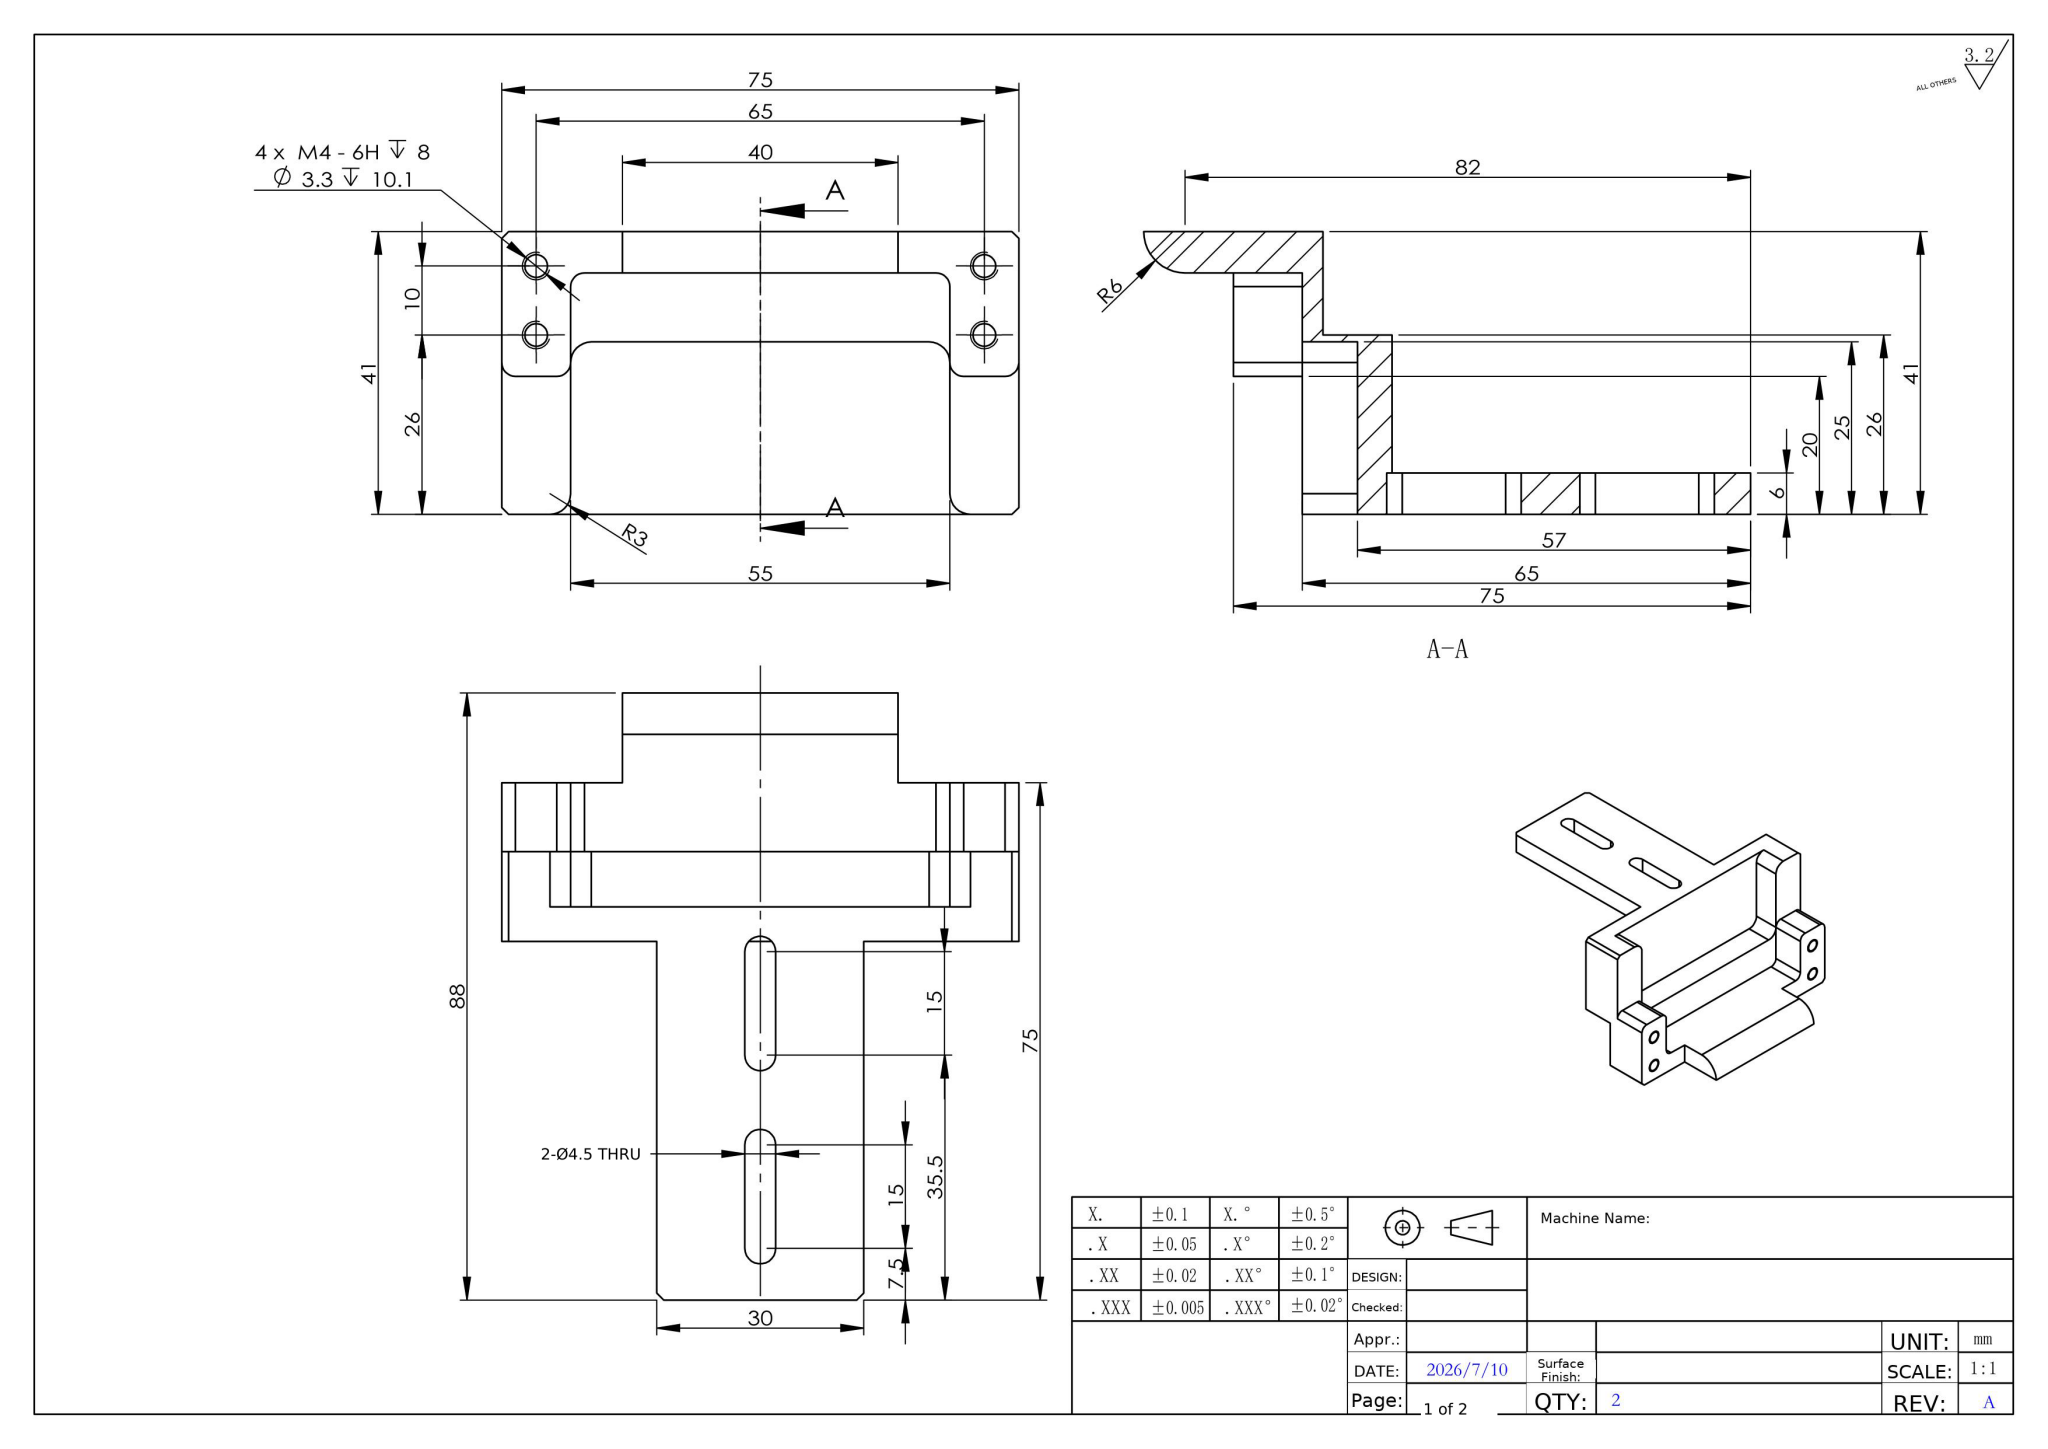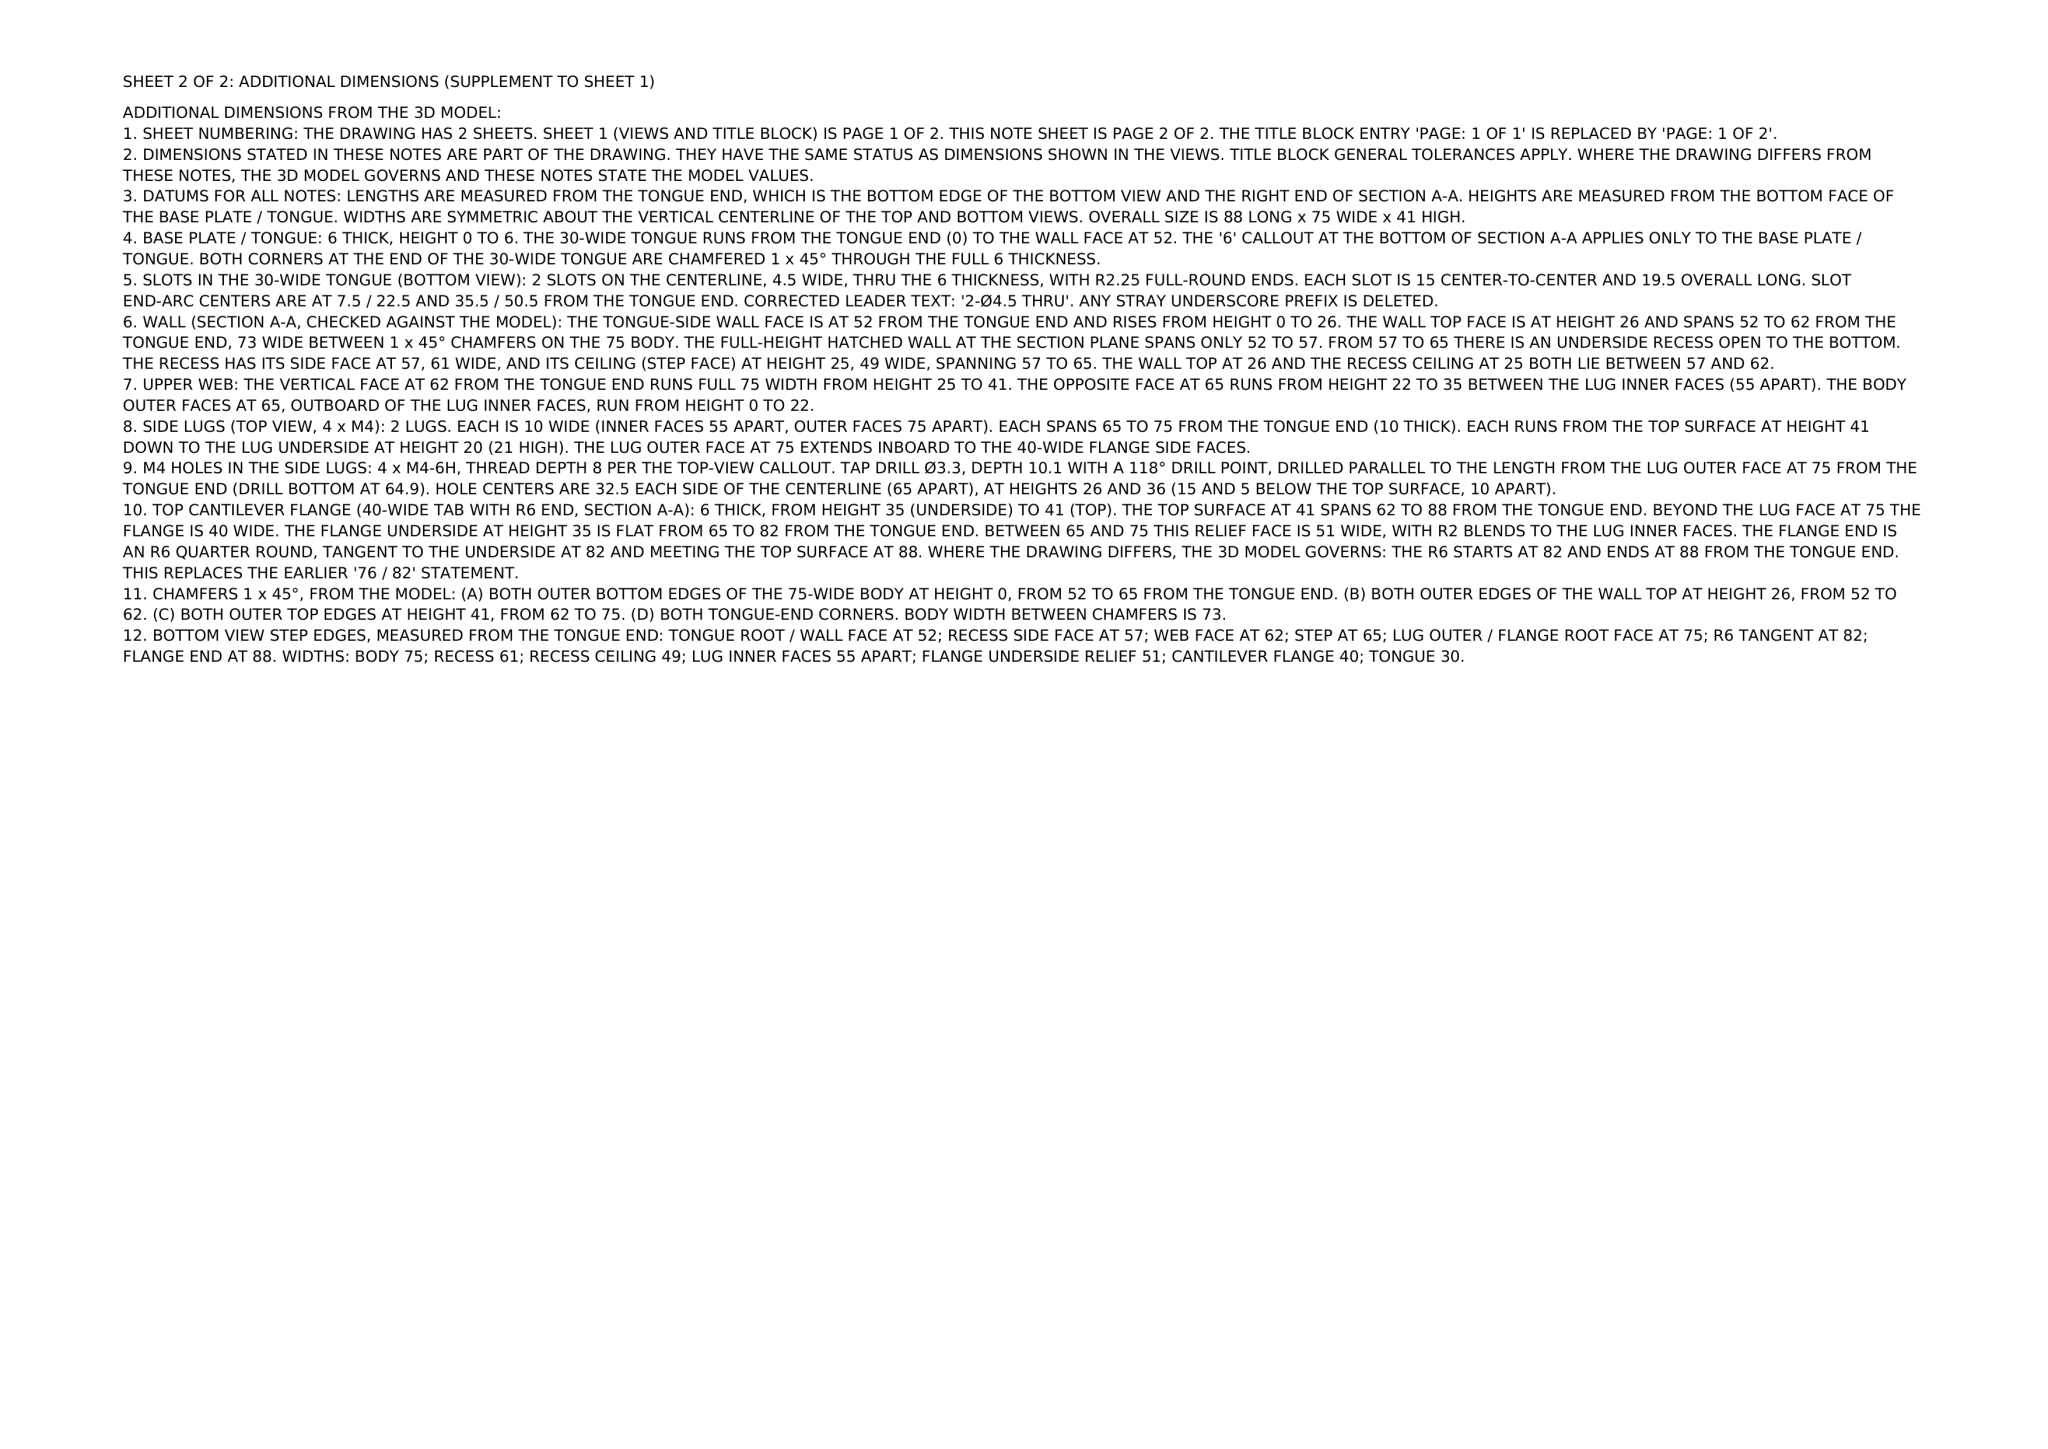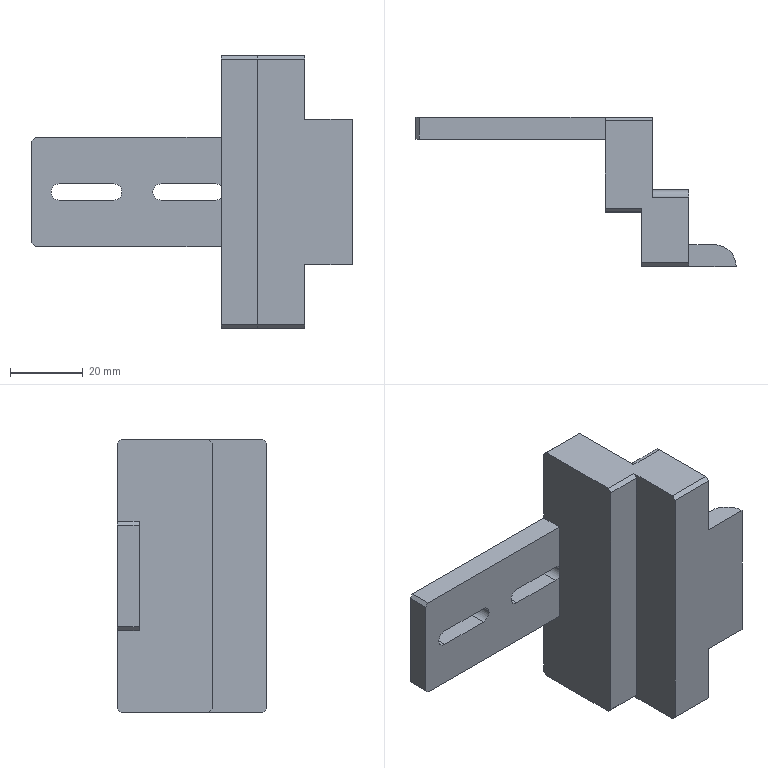Part | NX | mm | Slotted Corner Support Bracket | 1 solid | 73 faces | box 88 x 41 x 75 mm | volume 35979 mm3 | plane 40 | cylinder 25 | cone 8 | commonest cylinder face diameters 3.3 x8 4.5 x6 4 x6 6 x4 12 x1